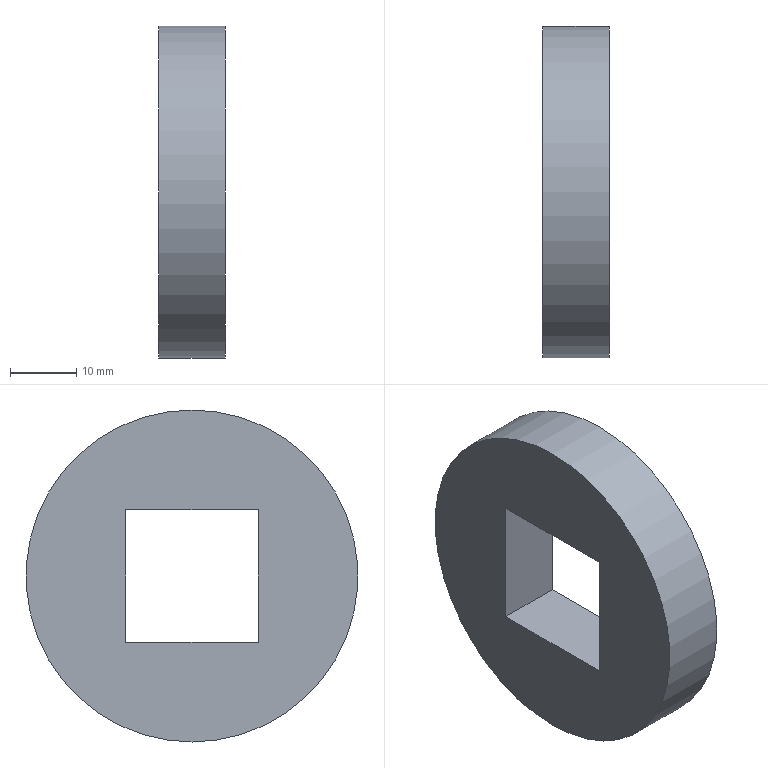Component | NX | FACEPLATE | 1 solid | 7 faces | box 10 x 50 x 50 mm | volume 15635 mm3 | plane 6 | cylinder 1 | commonest cylinder face diameters 50 x1
STEP:
#1=CARTESIAN_POINT('',(0.,0.,0.));
#2=DIRECTION('',(0.,0.,1.));
#3=DIRECTION('',(1.,0.,0.));
#4=AXIS2_PLACEMENT_3D('',#1,#2,#3);
#5=CARTESIAN_POINT('',(-39.,-10.,26.5));
#6=VERTEX_POINT('',#5);
#7=CARTESIAN_POINT('',(-39.,10.,26.5));
#8=VERTEX_POINT('',#7);
#9=CARTESIAN_POINT('',(-39.,-10.,26.5));
#10=DIRECTION('',(0.,1.,-0.));
#11=VECTOR('',#10,1.);
#12=LINE('',#9,#11);
#13=CARTESIAN_POINT('',(-49.,-10.,26.5));
#14=DIRECTION('',(0.,-0.,-1.));
#15=DIRECTION('',(0.,-1.,0.));
#16=AXIS2_PLACEMENT_3D('',#13,#14,#15);
#17=PLANE('',#16);
#18=CARTESIAN_POINT('',(0.,-10.));
#19=DIRECTION('',(-1.,0.));
#20=VECTOR('',#19,1.);
#21=LINE('',#18,#20);
#22=(GEOMETRIC_REPRESENTATION_CONTEXT(2)PARAMETRIC_REPRESENTATION_CONTEXT()REPRESENTATION_CONTEXT('',''));
#23=DEFINITIONAL_REPRESENTATION('',(#21),#22);
#24=PCURVE('',#17,#23);
#25=CARTESIAN_POINT('',(-39.,-0.,36.5));
#26=DIRECTION('',(-1.,0.,0.));
#27=DIRECTION('',(0.,0.,1.));
#28=AXIS2_PLACEMENT_3D('',#25,#26,#27);
#29=PLANE('',#28);
#30=CARTESIAN_POINT('',(-10.,-10.));
#31=DIRECTION('',(-0.,1.));
#32=VECTOR('',#31,1.);
#33=LINE('',#30,#32);
#34=(GEOMETRIC_REPRESENTATION_CONTEXT(2)PARAMETRIC_REPRESENTATION_CONTEXT()REPRESENTATION_CONTEXT('',''));
#35=DEFINITIONAL_REPRESENTATION('',(#33),#34);
#36=PCURVE('',#29,#35);
#37=SURFACE_CURVE('',#12,(#24,#36),.PCURVE_S1.);
#38=EDGE_CURVE('',#6,#8,#37,.T.);
#39=ORIENTED_EDGE('',*,*,#38,.T.);
#40=CARTESIAN_POINT('',(-49.,10.,26.5));
#41=VERTEX_POINT('',#40);
#42=CARTESIAN_POINT('',(-49.,10.,26.5));
#43=DIRECTION('',(1.,0.,0.));
#44=VECTOR('',#43,1.);
#45=LINE('',#42,#44);
#46=CARTESIAN_POINT('',(-20.,0.));
#47=DIRECTION('',(0.,-1.));
#48=VECTOR('',#47,1.);
#49=LINE('',#46,#48);
#50=(GEOMETRIC_REPRESENTATION_CONTEXT(2)PARAMETRIC_REPRESENTATION_CONTEXT()REPRESENTATION_CONTEXT('',''));
#51=DEFINITIONAL_REPRESENTATION('',(#49),#50);
#52=PCURVE('',#17,#51);
#53=CARTESIAN_POINT('',(-49.,10.,26.5));
#54=DIRECTION('',(0.,1.,0.));
#55=DIRECTION('',(-1.,0.,0.));
#56=AXIS2_PLACEMENT_3D('',#53,#54,#55);
#57=PLANE('',#56);
#58=CARTESIAN_POINT('',(0.,0.));
#59=DIRECTION('',(-1.,0.));
#60=VECTOR('',#59,1.);
#61=LINE('',#58,#60);
#62=(GEOMETRIC_REPRESENTATION_CONTEXT(2)PARAMETRIC_REPRESENTATION_CONTEXT()REPRESENTATION_CONTEXT('',''));
#63=DEFINITIONAL_REPRESENTATION('',(#61),#62);
#64=PCURVE('',#57,#63);
#65=SURFACE_CURVE('',#45,(#52,#64),.PCURVE_S1.);
#66=EDGE_CURVE('',#41,#8,#65,.T.);
#67=ORIENTED_EDGE('',*,*,#66,.F.);
#68=CARTESIAN_POINT('',(-49.,-10.,26.5));
#69=VERTEX_POINT('',#68);
#70=CARTESIAN_POINT('',(-49.,-10.,26.5));
#71=DIRECTION('',(0.,1.,-0.));
#72=VECTOR('',#71,1.);
#73=LINE('',#70,#72);
#74=CARTESIAN_POINT('',(0.,0.));
#75=DIRECTION('',(-1.,0.));
#76=VECTOR('',#75,1.);
#77=LINE('',#74,#76);
#78=(GEOMETRIC_REPRESENTATION_CONTEXT(2)PARAMETRIC_REPRESENTATION_CONTEXT()REPRESENTATION_CONTEXT('',''));
#79=DEFINITIONAL_REPRESENTATION('',(#77),#78);
#80=PCURVE('',#17,#79);
#81=CARTESIAN_POINT('',(-49.,-0.,36.5));
#82=DIRECTION('',(-1.,0.,0.));
#83=DIRECTION('',(0.,0.,1.));
#84=AXIS2_PLACEMENT_3D('',#81,#82,#83);
#85=PLANE('',#84);
#86=CARTESIAN_POINT('',(-10.,-10.));
#87=DIRECTION('',(-0.,1.));
#88=VECTOR('',#87,1.);
#89=LINE('',#86,#88);
#90=(GEOMETRIC_REPRESENTATION_CONTEXT(2)PARAMETRIC_REPRESENTATION_CONTEXT()REPRESENTATION_CONTEXT('',''));
#91=DEFINITIONAL_REPRESENTATION('',(#89),#90);
#92=PCURVE('',#85,#91);
#93=SURFACE_CURVE('',#73,(#80,#92),.PCURVE_S1.);
#94=EDGE_CURVE('',#69,#41,#93,.T.);
#95=ORIENTED_EDGE('',*,*,#94,.F.);
#96=CARTESIAN_POINT('',(-49.,-10.,26.5));
#97=DIRECTION('',(1.,0.,0.));
#98=VECTOR('',#97,1.);
#99=LINE('',#96,#98);
#100=CARTESIAN_POINT('',(0.,0.));
#101=DIRECTION('',(0.,-1.));
#102=VECTOR('',#101,1.);
#103=LINE('',#100,#102);
#104=(GEOMETRIC_REPRESENTATION_CONTEXT(2)PARAMETRIC_REPRESENTATION_CONTEXT()REPRESENTATION_CONTEXT('',''));
#105=DEFINITIONAL_REPRESENTATION('',(#103),#104);
#106=PCURVE('',#17,#105);
#107=CARTESIAN_POINT('',(-49.,-10.,46.5));
#108=DIRECTION('',(0.,-1.,0.));
#109=DIRECTION('',(0.,0.,1.));
#110=AXIS2_PLACEMENT_3D('',#107,#108,#109);
#111=PLANE('',#110);
#112=CARTESIAN_POINT('',(-20.,0.));
#113=DIRECTION('',(0.,-1.));
#114=VECTOR('',#113,1.);
#115=LINE('',#112,#114);
#116=(GEOMETRIC_REPRESENTATION_CONTEXT(2)PARAMETRIC_REPRESENTATION_CONTEXT()REPRESENTATION_CONTEXT('',''));
#117=DEFINITIONAL_REPRESENTATION('',(#115),#116);
#118=PCURVE('',#111,#117);
#119=SURFACE_CURVE('',#99,(#106,#118),.PCURVE_S1.);
#120=EDGE_CURVE('',#69,#6,#119,.T.);
#121=ORIENTED_EDGE('',*,*,#120,.T.);
#122=EDGE_LOOP('',(#39,#67,#95,#121));
#123=FACE_BOUND('',#122,.T.);
#124=ADVANCED_FACE('',(#123),#17,.F.);
#125=CARTESIAN_POINT('',(-39.,10.,46.5));
#126=VERTEX_POINT('',#125);
#127=CARTESIAN_POINT('',(-39.,10.,26.5));
#128=DIRECTION('',(0.,0.,1.));
#129=VECTOR('',#128,1.);
#130=LINE('',#127,#129);
#131=CARTESIAN_POINT('',(-10.,0.));
#132=DIRECTION('',(0.,1.));
#133=VECTOR('',#132,1.);
#134=LINE('',#131,#133);
#135=(GEOMETRIC_REPRESENTATION_CONTEXT(2)PARAMETRIC_REPRESENTATION_CONTEXT()REPRESENTATION_CONTEXT('',''));
#136=DEFINITIONAL_REPRESENTATION('',(#134),#135);
#137=PCURVE('',#57,#136);
#138=CARTESIAN_POINT('',(-10.,10.));
#139=DIRECTION('',(1.,0.));
#140=VECTOR('',#139,1.);
#141=LINE('',#138,#140);
#142=(GEOMETRIC_REPRESENTATION_CONTEXT(2)PARAMETRIC_REPRESENTATION_CONTEXT()REPRESENTATION_CONTEXT('',''));
#143=DEFINITIONAL_REPRESENTATION('',(#141),#142);
#144=PCURVE('',#29,#143);
#145=SURFACE_CURVE('',#130,(#137,#144),.PCURVE_S1.);
#146=EDGE_CURVE('',#8,#126,#145,.T.);
#147=ORIENTED_EDGE('',*,*,#146,.T.);
#148=CARTESIAN_POINT('',(-49.,10.,46.5));
#149=VERTEX_POINT('',#148);
#150=CARTESIAN_POINT('',(-49.,10.,46.5));
#151=DIRECTION('',(1.,0.,0.));
#152=VECTOR('',#151,1.);
#153=LINE('',#150,#152);
#154=CARTESIAN_POINT('',(0.,20.));
#155=DIRECTION('',(-1.,0.));
#156=VECTOR('',#155,1.);
#157=LINE('',#154,#156);
#158=(GEOMETRIC_REPRESENTATION_CONTEXT(2)PARAMETRIC_REPRESENTATION_CONTEXT()REPRESENTATION_CONTEXT('',''));
#159=DEFINITIONAL_REPRESENTATION('',(#157),#158);
#160=PCURVE('',#57,#159);
#161=CARTESIAN_POINT('',(-49.,10.,46.5));
#162=DIRECTION('',(0.,0.,1.));
#163=DIRECTION('',(0.,1.,-0.));
#164=AXIS2_PLACEMENT_3D('',#161,#162,#163);
#165=PLANE('',#164);
#166=CARTESIAN_POINT('',(0.,0.));
#167=DIRECTION('',(0.,-1.));
#168=VECTOR('',#167,1.);
#169=LINE('',#166,#168);
#170=(GEOMETRIC_REPRESENTATION_CONTEXT(2)PARAMETRIC_REPRESENTATION_CONTEXT()REPRESENTATION_CONTEXT('',''));
#171=DEFINITIONAL_REPRESENTATION('',(#169),#170);
#172=PCURVE('',#165,#171);
#173=SURFACE_CURVE('',#153,(#160,#172),.PCURVE_S1.);
#174=EDGE_CURVE('',#149,#126,#173,.T.);
#175=ORIENTED_EDGE('',*,*,#174,.F.);
#176=CARTESIAN_POINT('',(-49.,10.,26.5));
#177=DIRECTION('',(0.,0.,1.));
#178=VECTOR('',#177,1.);
#179=LINE('',#176,#178);
#180=CARTESIAN_POINT('',(0.,0.));
#181=DIRECTION('',(0.,1.));
#182=VECTOR('',#181,1.);
#183=LINE('',#180,#182);
#184=(GEOMETRIC_REPRESENTATION_CONTEXT(2)PARAMETRIC_REPRESENTATION_CONTEXT()REPRESENTATION_CONTEXT('',''));
#185=DEFINITIONAL_REPRESENTATION('',(#183),#184);
#186=PCURVE('',#57,#185);
#187=CARTESIAN_POINT('',(-10.,10.));
#188=DIRECTION('',(1.,0.));
#189=VECTOR('',#188,1.);
#190=LINE('',#187,#189);
#191=(GEOMETRIC_REPRESENTATION_CONTEXT(2)PARAMETRIC_REPRESENTATION_CONTEXT()REPRESENTATION_CONTEXT('',''));
#192=DEFINITIONAL_REPRESENTATION('',(#190),#191);
#193=PCURVE('',#85,#192);
#194=SURFACE_CURVE('',#179,(#186,#193),.PCURVE_S1.);
#195=EDGE_CURVE('',#41,#149,#194,.T.);
#196=ORIENTED_EDGE('',*,*,#195,.F.);
#197=ORIENTED_EDGE('',*,*,#66,.T.);
#198=EDGE_LOOP('',(#147,#175,#196,#197));
#199=FACE_BOUND('',#198,.T.);
#200=ADVANCED_FACE('',(#199),#57,.F.);
#201=CARTESIAN_POINT('',(-39.,-10.,46.5));
#202=VERTEX_POINT('',#201);
#203=CARTESIAN_POINT('',(-39.,10.,46.5));
#204=DIRECTION('',(0.,-1.,0.));
#205=VECTOR('',#204,1.);
#206=LINE('',#203,#205);
#207=CARTESIAN_POINT('',(0.,-10.));
#208=DIRECTION('',(-1.,0.));
#209=VECTOR('',#208,1.);
#210=LINE('',#207,#209);
#211=(GEOMETRIC_REPRESENTATION_CONTEXT(2)PARAMETRIC_REPRESENTATION_CONTEXT()REPRESENTATION_CONTEXT('',''));
#212=DEFINITIONAL_REPRESENTATION('',(#210),#211);
#213=PCURVE('',#165,#212);
#214=CARTESIAN_POINT('',(10.,10.));
#215=DIRECTION('',(0.,-1.));
#216=VECTOR('',#215,1.);
#217=LINE('',#214,#216);
#218=(GEOMETRIC_REPRESENTATION_CONTEXT(2)PARAMETRIC_REPRESENTATION_CONTEXT()REPRESENTATION_CONTEXT('',''));
#219=DEFINITIONAL_REPRESENTATION('',(#217),#218);
#220=PCURVE('',#29,#219);
#221=SURFACE_CURVE('',#206,(#213,#220),.PCURVE_S1.);
#222=EDGE_CURVE('',#126,#202,#221,.T.);
#223=ORIENTED_EDGE('',*,*,#222,.T.);
#224=CARTESIAN_POINT('',(-49.,-10.,46.5));
#225=VERTEX_POINT('',#224);
#226=CARTESIAN_POINT('',(-49.,-10.,46.5));
#227=DIRECTION('',(1.,0.,0.));
#228=VECTOR('',#227,1.);
#229=LINE('',#226,#228);
#230=CARTESIAN_POINT('',(-20.,0.));
#231=DIRECTION('',(0.,-1.));
#232=VECTOR('',#231,1.);
#233=LINE('',#230,#232);
#234=(GEOMETRIC_REPRESENTATION_CONTEXT(2)PARAMETRIC_REPRESENTATION_CONTEXT()REPRESENTATION_CONTEXT('',''));
#235=DEFINITIONAL_REPRESENTATION('',(#233),#234);
#236=PCURVE('',#165,#235);
#237=CARTESIAN_POINT('',(0.,0.));
#238=DIRECTION('',(0.,-1.));
#239=VECTOR('',#238,1.);
#240=LINE('',#237,#239);
#241=(GEOMETRIC_REPRESENTATION_CONTEXT(2)PARAMETRIC_REPRESENTATION_CONTEXT()REPRESENTATION_CONTEXT('',''));
#242=DEFINITIONAL_REPRESENTATION('',(#240),#241);
#243=PCURVE('',#111,#242);
#244=SURFACE_CURVE('',#229,(#236,#243),.PCURVE_S1.);
#245=EDGE_CURVE('',#225,#202,#244,.T.);
#246=ORIENTED_EDGE('',*,*,#245,.F.);
#247=CARTESIAN_POINT('',(-49.,10.,46.5));
#248=DIRECTION('',(0.,-1.,0.));
#249=VECTOR('',#248,1.);
#250=LINE('',#247,#249);
#251=CARTESIAN_POINT('',(0.,0.));
#252=DIRECTION('',(-1.,0.));
#253=VECTOR('',#252,1.);
#254=LINE('',#251,#253);
#255=(GEOMETRIC_REPRESENTATION_CONTEXT(2)PARAMETRIC_REPRESENTATION_CONTEXT()REPRESENTATION_CONTEXT('',''));
#256=DEFINITIONAL_REPRESENTATION('',(#254),#255);
#257=PCURVE('',#165,#256);
#258=CARTESIAN_POINT('',(10.,10.));
#259=DIRECTION('',(0.,-1.));
#260=VECTOR('',#259,1.);
#261=LINE('',#258,#260);
#262=(GEOMETRIC_REPRESENTATION_CONTEXT(2)PARAMETRIC_REPRESENTATION_CONTEXT()REPRESENTATION_CONTEXT('',''));
#263=DEFINITIONAL_REPRESENTATION('',(#261),#262);
#264=PCURVE('',#85,#263);
#265=SURFACE_CURVE('',#250,(#257,#264),.PCURVE_S1.);
#266=EDGE_CURVE('',#149,#225,#265,.T.);
#267=ORIENTED_EDGE('',*,*,#266,.F.);
#268=ORIENTED_EDGE('',*,*,#174,.T.);
#269=EDGE_LOOP('',(#223,#246,#267,#268));
#270=FACE_BOUND('',#269,.T.);
#271=ADVANCED_FACE('',(#270),#165,.F.);
#272=CARTESIAN_POINT('',(-49.,-0.,61.5));
#273=VERTEX_POINT('',#272);
#274=CARTESIAN_POINT('',(-49.,-0.,36.5));
#275=DIRECTION('',(-1.,0.,0.));
#276=DIRECTION('',(0.,0.,1.));
#277=AXIS2_PLACEMENT_3D('',#274,#275,#276);
#278=CIRCLE('',#277,25.);
#279=CARTESIAN_POINT('',(-49.,-0.,36.5));
#280=DIRECTION('',(1.,0.,0.));
#281=DIRECTION('',(0.,0.,-1.));
#282=AXIS2_PLACEMENT_3D('',#279,#280,#281);
#283=CYLINDRICAL_SURFACE('',#282,25.);
#284=CARTESIAN_POINT('',(9.425,0.));
#285=DIRECTION('',(-1.,0.));
#286=VECTOR('',#285,1.);
#287=LINE('',#284,#286);
#288=(GEOMETRIC_REPRESENTATION_CONTEXT(2)PARAMETRIC_REPRESENTATION_CONTEXT()REPRESENTATION_CONTEXT('',''));
#289=DEFINITIONAL_REPRESENTATION('',(#287),#288);
#290=PCURVE('',#283,#289);
#291=CARTESIAN_POINT('',(0.,0.));
#292=DIRECTION('',(1.,0.));
#293=AXIS2_PLACEMENT_2D('',#291,#292);
#294=CIRCLE('',#293,25.);
#295=(GEOMETRIC_REPRESENTATION_CONTEXT(2)PARAMETRIC_REPRESENTATION_CONTEXT()REPRESENTATION_CONTEXT('',''));
#296=DEFINITIONAL_REPRESENTATION('',(#294),#295);
#297=PCURVE('',#85,#296);
#298=SURFACE_CURVE('',#278,(#290,#297),.PCURVE_S1.);
#299=EDGE_CURVE('',#273,#273,#298,.T.);
#300=ORIENTED_EDGE('',*,*,#299,.F.);
#301=CARTESIAN_POINT('',(-39.,-0.,61.5));
#302=VERTEX_POINT('',#301);
#303=CARTESIAN_POINT('',(-49.,0.,61.5));
#304=CARTESIAN_POINT('',(-39.,0.,61.5));
#305=B_SPLINE_CURVE_WITH_KNOTS('',1,(#303,#304),.UNSPECIFIED.,.F.,.F.,(2,2),(0.,10.),.PIECEWISE_BEZIER_KNOTS.);
#306=CARTESIAN_POINT('',(9.425,0.));
#307=DIRECTION('',(0.,1.));
#308=VECTOR('',#307,1.);
#309=LINE('',#306,#308);
#310=(GEOMETRIC_REPRESENTATION_CONTEXT(2)PARAMETRIC_REPRESENTATION_CONTEXT()REPRESENTATION_CONTEXT('',''));
#311=DEFINITIONAL_REPRESENTATION('',(#309),#310);
#312=PCURVE('',#283,#311);
#313=CARTESIAN_POINT('',(3.142,0.));
#314=DIRECTION('',(0.,1.));
#315=VECTOR('',#314,1.);
#316=LINE('',#313,#315);
#317=(GEOMETRIC_REPRESENTATION_CONTEXT(2)PARAMETRIC_REPRESENTATION_CONTEXT()REPRESENTATION_CONTEXT('',''));
#318=DEFINITIONAL_REPRESENTATION('',(#316),#317);
#319=PCURVE('',#283,#318);
#320=SEAM_CURVE('',#305,(#312,#319),.PCURVE_S1.);
#321=EDGE_CURVE('',#273,#302,#320,.T.);
#322=ORIENTED_EDGE('',*,*,#321,.T.);
#323=CARTESIAN_POINT('',(-39.,-0.,36.5));
#324=DIRECTION('',(-1.,0.,0.));
#325=DIRECTION('',(0.,0.,1.));
#326=AXIS2_PLACEMENT_3D('',#323,#324,#325);
#327=CIRCLE('',#326,25.);
#328=CARTESIAN_POINT('',(9.425,10.));
#329=DIRECTION('',(-1.,0.));
#330=VECTOR('',#329,1.);
#331=LINE('',#328,#330);
#332=(GEOMETRIC_REPRESENTATION_CONTEXT(2)PARAMETRIC_REPRESENTATION_CONTEXT()REPRESENTATION_CONTEXT('',''));
#333=DEFINITIONAL_REPRESENTATION('',(#331),#332);
#334=PCURVE('',#283,#333);
#335=CARTESIAN_POINT('',(0.,0.));
#336=DIRECTION('',(1.,0.));
#337=AXIS2_PLACEMENT_2D('',#335,#336);
#338=CIRCLE('',#337,25.);
#339=(GEOMETRIC_REPRESENTATION_CONTEXT(2)PARAMETRIC_REPRESENTATION_CONTEXT()REPRESENTATION_CONTEXT('',''));
#340=DEFINITIONAL_REPRESENTATION('',(#338),#339);
#341=PCURVE('',#29,#340);
#342=SURFACE_CURVE('',#327,(#334,#341),.PCURVE_S1.);
#343=EDGE_CURVE('',#302,#302,#342,.T.);
#344=ORIENTED_EDGE('',*,*,#343,.T.);
#345=ORIENTED_EDGE('',*,*,#321,.F.);
#346=EDGE_LOOP('',(#300,#322,#344,#345));
#347=FACE_BOUND('',#346,.T.);
#348=ADVANCED_FACE('',(#347),#283,.T.);
#349=CARTESIAN_POINT('',(-39.,-10.,46.5));
#350=DIRECTION('',(0.,-0.,-1.));
#351=VECTOR('',#350,1.);
#352=LINE('',#349,#351);
#353=CARTESIAN_POINT('',(0.,-10.));
#354=DIRECTION('',(-1.,0.));
#355=VECTOR('',#354,1.);
#356=LINE('',#353,#355);
#357=(GEOMETRIC_REPRESENTATION_CONTEXT(2)PARAMETRIC_REPRESENTATION_CONTEXT()REPRESENTATION_CONTEXT('',''));
#358=DEFINITIONAL_REPRESENTATION('',(#356),#357);
#359=PCURVE('',#111,#358);
#360=CARTESIAN_POINT('',(10.,-10.));
#361=DIRECTION('',(-1.,-0.));
#362=VECTOR('',#361,1.);
#363=LINE('',#360,#362);
#364=(GEOMETRIC_REPRESENTATION_CONTEXT(2)PARAMETRIC_REPRESENTATION_CONTEXT()REPRESENTATION_CONTEXT('',''));
#365=DEFINITIONAL_REPRESENTATION('',(#363),#364);
#366=PCURVE('',#29,#365);
#367=SURFACE_CURVE('',#352,(#359,#366),.PCURVE_S1.);
#368=EDGE_CURVE('',#202,#6,#367,.T.);
#369=ORIENTED_EDGE('',*,*,#368,.T.);
#370=ORIENTED_EDGE('',*,*,#120,.F.);
#371=CARTESIAN_POINT('',(-49.,-10.,46.5));
#372=DIRECTION('',(0.,-0.,-1.));
#373=VECTOR('',#372,1.);
#374=LINE('',#371,#373);
#375=CARTESIAN_POINT('',(0.,0.));
#376=DIRECTION('',(-1.,0.));
#377=VECTOR('',#376,1.);
#378=LINE('',#375,#377);
#379=(GEOMETRIC_REPRESENTATION_CONTEXT(2)PARAMETRIC_REPRESENTATION_CONTEXT()REPRESENTATION_CONTEXT('',''));
#380=DEFINITIONAL_REPRESENTATION('',(#378),#379);
#381=PCURVE('',#111,#380);
#382=CARTESIAN_POINT('',(10.,-10.));
#383=DIRECTION('',(-1.,-0.));
#384=VECTOR('',#383,1.);
#385=LINE('',#382,#384);
#386=(GEOMETRIC_REPRESENTATION_CONTEXT(2)PARAMETRIC_REPRESENTATION_CONTEXT()REPRESENTATION_CONTEXT('',''));
#387=DEFINITIONAL_REPRESENTATION('',(#385),#386);
#388=PCURVE('',#85,#387);
#389=SURFACE_CURVE('',#374,(#381,#388),.PCURVE_S1.);
#390=EDGE_CURVE('',#225,#69,#389,.T.);
#391=ORIENTED_EDGE('',*,*,#390,.F.);
#392=ORIENTED_EDGE('',*,*,#245,.T.);
#393=EDGE_LOOP('',(#369,#370,#391,#392));
#394=FACE_BOUND('',#393,.T.);
#395=ADVANCED_FACE('',(#394),#111,.F.);
#396=ORIENTED_EDGE('',*,*,#299,.T.);
#397=EDGE_LOOP('',(#396));
#398=FACE_BOUND('',#397,.T.);
#399=ORIENTED_EDGE('',*,*,#94,.T.);
#400=ORIENTED_EDGE('',*,*,#195,.T.);
#401=ORIENTED_EDGE('',*,*,#266,.T.);
#402=ORIENTED_EDGE('',*,*,#390,.T.);
#403=EDGE_LOOP('',(#399,#400,#401,#402));
#404=FACE_BOUND('',#403,.T.);
#405=ADVANCED_FACE('',(#398,#404),#85,.T.);
#406=ORIENTED_EDGE('',*,*,#343,.F.);
#407=EDGE_LOOP('',(#406));
#408=FACE_BOUND('',#407,.T.);
#409=ORIENTED_EDGE('',*,*,#38,.F.);
#410=ORIENTED_EDGE('',*,*,#368,.F.);
#411=ORIENTED_EDGE('',*,*,#222,.F.);
#412=ORIENTED_EDGE('',*,*,#146,.F.);
#413=EDGE_LOOP('',(#409,#410,#411,#412));
#414=FACE_BOUND('',#413,.T.);
#415=ADVANCED_FACE('',(#408,#414),#29,.F.);
#416=CLOSED_SHELL('',(#124,#200,#271,#348,#395,#405,#415));
#417=MANIFOLD_SOLID_BREP('',#416);
#418=(LENGTH_UNIT()NAMED_UNIT(*)SI_UNIT(.MILLI.,.METRE.));
#419=UNCERTAINTY_MEASURE_WITH_UNIT(LENGTH_MEASURE(0.000002),#418,'','');
#420=(NAMED_UNIT(*)PLANE_ANGLE_UNIT()SI_UNIT($,.RADIAN.));
#421=(NAMED_UNIT(*)SI_UNIT($,.STERADIAN.)SOLID_ANGLE_UNIT());
#422=(GEOMETRIC_REPRESENTATION_CONTEXT(3)GLOBAL_UNCERTAINTY_ASSIGNED_CONTEXT((#419))GLOBAL_UNIT_ASSIGNED_CONTEXT((#418,#420,#421))REPRESENTATION_CONTEXT('',''));
#423=ADVANCED_BREP_SHAPE_REPRESENTATION('',(#4,#417),#422);